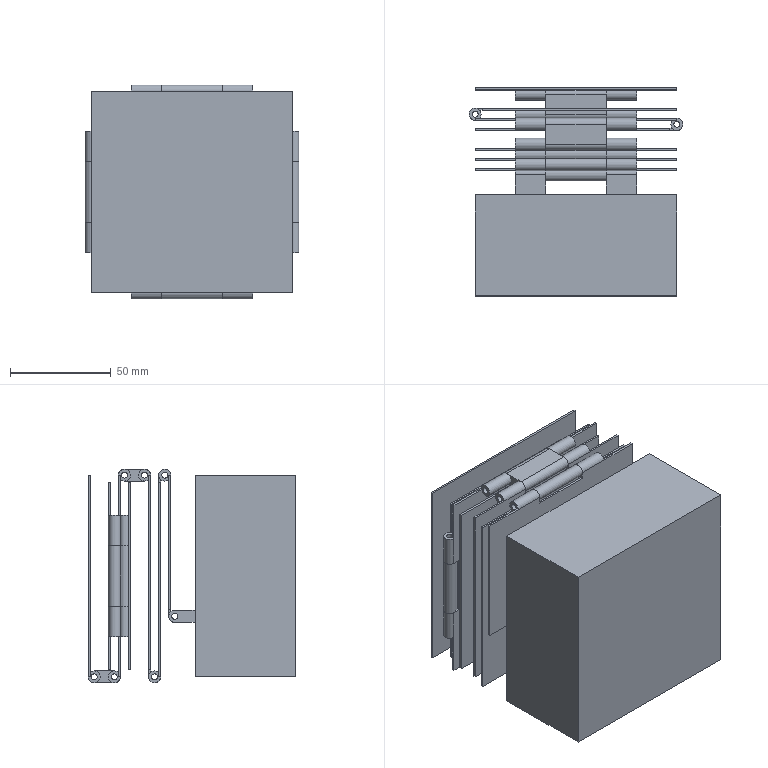Assembly | NX | mm | 10 component files | 10 solids | 181 faces | box 106 x 103 x 106 mm | volume 577711 mm3 | plane 127 | cylinder 54 | commonest cylinder face diameters 6 x27 3 x27
Bill of materials:
unnamed part 1 | 1 |  | Thin flat square plate with two rolled cylindrical knuckles (hollow, with bores) on each of its four edges, eight knuckles in total. Each one sits in a notch or offset step along the edge.
unnamed part 2 | 2 |  | Thin flat rectangular plate with one hollow cylindrical knuckle along part of one edge.
unnamed part 3 | 2 |  | Thin flat rectangular plate with two short hollow knuckles on one edge and one longer hollow knuckle on the opposite edge. The knuckles on the two edges are staggered.
unnamed part 4 | 1 |  | Rectangular block-like solid. Two of the orthographic views also show two tabs projecting from one face and a small tab with a hole (eyelet-like) projecting from another face.
unnamed part 5 | 2 |  | Straight prismatic bar with an obround (stadium-shaped) cross-section and two parallel round through-holes along its full length, one near each rounded end.
unnamed part 6 | 1 |  | Thin flat square plate with two short hollow cylindrical knuckles on one edge, separated by a notch in the plate edge.
unnamed part 7 | 1 |  | Thin flat rectangular plate, wider than it is tall, with two short hollow knuckles on one long edge and one longer centered hollow knuckle on the opposite long edge. The knuckles are staggered.
Mates:
1. fix | part_1 1 component
2. concentric | part_2 1 edge | part_1 1 edge
3. concentric | part_3 2 edge | part_2 1 edge
4. concentric | part_3 1 edge | part_3 2 edge
5. concentric | part_4 2 edge | part_3 1 edge
6. concentric | part_5 1 edge | part_4 2 edge
7. concentric | part_4 1 edge | part_5 1 edge
8. concentric | part_6 2 edge | part_5 1 edge
9. concentric | part_6 1 edge | part_5 1 edge
10. concentric | part_7 1 edge | part_4 1 edge